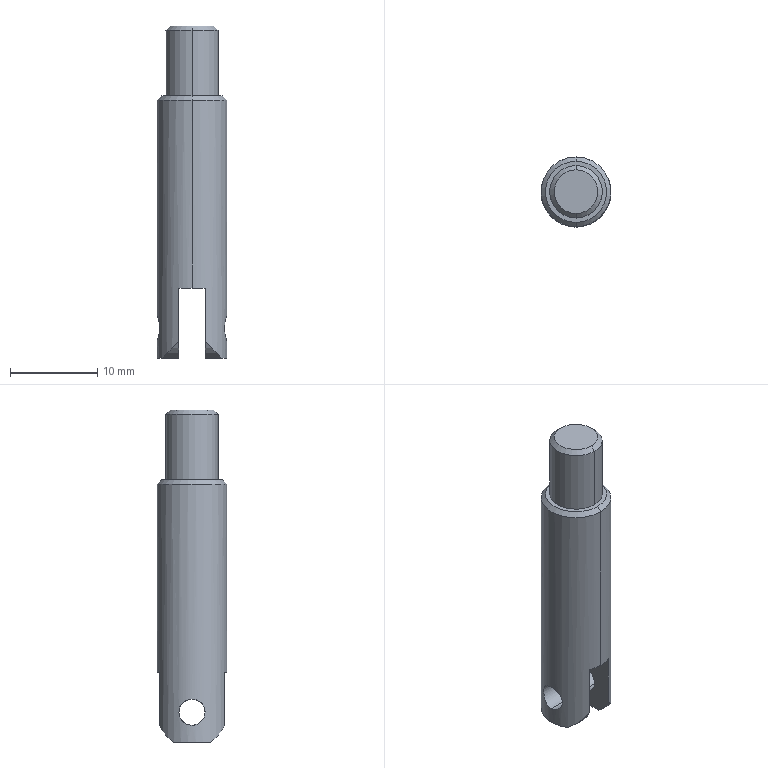Component | SolidWorks | GuideRod1-1 | 1 solid | 23 faces | box 8 x 8 x 38 mm | volume 1503 mm3 | cylinder 12 | plane 7 | cone 4 | commonest cylinder face diameters 8 x6 3 x4 6 x2
build123d program:
from build123d import *

# Parameters (mm, degrees)
SKETCH1_R           = 4
BOSS_EXTRUDE1_DEPTH = 30
SKETCH2_R           = 3
BOSS_EXTRUDE2_DEPTH = 8
CUT_EXTRUDE1_DEPTH  = 13
SKETCH5_W           = 16
SKETCH5_H           = 3
CUT_EXTRUDE2_DEPTH  = 13
SKETCH6_R           = 1.5
CUT_EXTRUDE3_DEPTH  = 13
CHAMFER1_SIZE       = 0.5


with BuildPart() as part:
    # Sketch1 → Boss-Extrude1 (new body)
    with BuildSketch(Plane.XY):
        Circle(SKETCH1_R)
    extrude(amount=BOSS_EXTRUDE1_DEPTH)

    # Sketch2 → Boss-Extrude2 (add)
    with BuildSketch(Plane(origin=(0, 0, 0), x_dir=(-1, 0, 0), z_dir=(0, 0, -1))):
        with Locations(Location((0, 0, 0), (0, 0, 180))):
            Circle(SKETCH2_R)
    extrude(amount=BOSS_EXTRUDE2_DEPTH)

    # Sketch4 → Cut-Extrude1 (cut, symmetric)
    with BuildSketch(Plane(origin=(0, 0, 0), x_dir=(1, 0, 0), z_dir=(0, 1, 0))):
        with BuildLine():
            Line((-4, -26.584), (-9.687, -26.584))
            Line((-9.687, -26.584), (-6.844, -32.06))
            Line((-6.844, -32.06), (5.728, -32.06))
            Line((5.728, -32.06), (7.666, -26.584))
            Line((7.666, -26.584), (4, -26.584))
            ThreePointArc((4, -26.584), (0, -30.584), (-4, -26.584))
        make_face()
    extrude(amount=CUT_EXTRUDE1_DEPTH, both=True, mode=Mode.SUBTRACT)

    # Sketch5 → Cut-Extrude2 (cut, symmetric)
    with BuildSketch(Plane(origin=(0, 0, 0), x_dir=(0, 0, -1), z_dir=(1, 0, 0))):
        with Locations((-30, 0)):
            Rectangle(SKETCH5_W, SKETCH5_H)
    extrude(amount=CUT_EXTRUDE2_DEPTH, both=True, mode=Mode.SUBTRACT)

    # Sketch6 → Cut-Extrude3 (cut, symmetric)
    with BuildSketch(Plane(origin=(0, 0, 0), x_dir=(1, 0, 0), z_dir=(0, 1, 0))):
        with Locations(Location((0, -26.584, 0), (0, 0, 270))):
            Circle(SKETCH6_R)
    extrude(amount=CUT_EXTRUDE3_DEPTH, both=True, mode=Mode.SUBTRACT)

    # Chamfer1
    chamfer1_edges = [part.edges().sort_by_distance(p)[0] for p in [
        (-4, 0, 0),
        (-3, 0, -8),
    ]]
    chamfer(chamfer1_edges, length=CHAMFER1_SIZE)


solid = part.part

# Placed as in the assembly
solid = solid.moved(Location((-15.928, -1.7, 62), (180, 0, -90)))
STEP:
#1=COLOUR_RGB('',0.7922,0.8196,0.9333);
#2=FILL_AREA_STYLE_COLOUR('',#1);
#3=FILL_AREA_STYLE('',(#2));
#4=SURFACE_STYLE_FILL_AREA(#3);
#5=SURFACE_SIDE_STYLE('',(#4));
#6=SURFACE_STYLE_USAGE(.BOTH.,#5);
#7=PRESENTATION_STYLE_ASSIGNMENT((#6));
#8=CARTESIAN_POINT('',(-0.6271,-0.1654,2.756));
#9=VERTEX_POINT('',#8);
#10=CARTESIAN_POINT('',(-0.6271,0.03149,2.756));
#11=VERTEX_POINT('',#10);
#12=CARTESIAN_POINT('',(-0.6271,-0.06694,2.756));
#13=DIRECTION('',(0.,0.,1.));
#14=DIRECTION('',(0.,-1.,0.));
#15=AXIS2_PLACEMENT_3D('',#12,#13,#14);
#16=CIRCLE('',#15,0.09843);
#17=EDGE_CURVE('',#9,#11,#16,.T.);
#18=ORIENTED_EDGE('',*,*,#17,.F.);
#19=CARTESIAN_POINT('',(-0.6271,-0.185,2.736));
#20=VERTEX_POINT('',#19);
#21=CARTESIAN_POINT('',(-0.6271,-0.1654,2.756));
#22=DIRECTION('',(0.,-0.7071,-0.7071));
#23=VECTOR('',#22,39.37);
#24=LINE('',#21,#23);
#25=EDGE_CURVE('',#9,#20,#24,.T.);
#26=ORIENTED_EDGE('',*,*,#25,.T.);
#27=CARTESIAN_POINT('',(-0.6271,0.05117,2.736));
#28=VERTEX_POINT('',#27);
#29=CARTESIAN_POINT('',(-0.6271,-0.06694,2.736));
#30=DIRECTION('',(0.,0.,-1.));
#31=DIRECTION('',(0.,-1.,0.));
#32=AXIS2_PLACEMENT_3D('',#29,#30,#31);
#33=CIRCLE('',#32,0.1181);
#34=EDGE_CURVE('',#28,#20,#33,.T.);
#35=ORIENTED_EDGE('',*,*,#34,.F.);
#36=CARTESIAN_POINT('',(-0.6271,0.03149,2.756));
#37=DIRECTION('',(-0.,0.7071,-0.7071));
#38=VECTOR('',#37,39.37);
#39=LINE('',#36,#38);
#40=EDGE_CURVE('',#11,#28,#39,.T.);
#41=ORIENTED_EDGE('',*,*,#40,.F.);
#42=EDGE_LOOP('',(#18,#26,#35,#41));
#43=FACE_OUTER_BOUND('',#42,.T.);
#44=CARTESIAN_POINT('',(-0.6271,-0.06694,2.756));
#45=DIRECTION('',(0.,0.,-1.));
#46=DIRECTION('',(0.,1.,0.));
#47=AXIS2_PLACEMENT_3D('',#44,#45,#46);
#48=CONICAL_SURFACE('',#47,0.09843,0.7854);
#49=ADVANCED_FACE('',(#43),#48,.T.);
#50=CARTESIAN_POINT('',(-0.6271,-0.2047,2.441));
#51=VERTEX_POINT('',#50);
#52=CARTESIAN_POINT('',(-0.6271,0.07086,2.441));
#53=VERTEX_POINT('',#52);
#54=CARTESIAN_POINT('',(-0.6271,-0.06694,2.441));
#55=DIRECTION('',(0.,0.,1.));
#56=DIRECTION('',(0.,1.,0.));
#57=AXIS2_PLACEMENT_3D('',#54,#55,#56);
#58=CIRCLE('',#57,0.1378);
#59=EDGE_CURVE('',#51,#53,#58,.T.);
#60=ORIENTED_EDGE('',*,*,#59,.F.);
#61=CARTESIAN_POINT('',(-0.6271,-0.2244,2.421));
#62=VERTEX_POINT('',#61);
#63=CARTESIAN_POINT('',(-0.6271,-0.2244,2.421));
#64=DIRECTION('',(0.,-0.7071,-0.7071));
#65=VECTOR('',#64,39.37);
#66=LINE('',#63,#65);
#67=EDGE_CURVE('',#51,#62,#66,.T.);
#68=ORIENTED_EDGE('',*,*,#67,.T.);
#69=CARTESIAN_POINT('',(-0.6271,0.09054,2.421));
#70=VERTEX_POINT('',#69);
#71=CARTESIAN_POINT('',(-0.6271,-0.06694,2.421));
#72=DIRECTION('',(0.,0.,-1.));
#73=DIRECTION('',(0.,1.,0.));
#74=AXIS2_PLACEMENT_3D('',#71,#72,#73);
#75=CIRCLE('',#74,0.1575);
#76=EDGE_CURVE('',#70,#62,#75,.T.);
#77=ORIENTED_EDGE('',*,*,#76,.F.);
#78=CARTESIAN_POINT('',(-0.6271,0.09054,2.421));
#79=DIRECTION('',(-0.,0.7071,-0.7071));
#80=VECTOR('',#79,39.37);
#81=LINE('',#78,#80);
#82=EDGE_CURVE('',#53,#70,#81,.T.);
#83=ORIENTED_EDGE('',*,*,#82,.F.);
#84=EDGE_LOOP('',(#60,#68,#77,#83));
#85=FACE_OUTER_BOUND('',#84,.T.);
#86=CARTESIAN_POINT('',(-0.6271,-0.06694,2.421));
#87=DIRECTION('',(0.,0.,-1.));
#88=DIRECTION('',(0.,1.,0.));
#89=AXIS2_PLACEMENT_3D('',#86,#87,#88);
#90=CONICAL_SURFACE('',#89,0.1575,0.7854);
#91=ADVANCED_FACE('',(#85),#90,.T.);
#92=CARTESIAN_POINT('',(-0.7846,-0.06694,1.453));
#93=VERTEX_POINT('',#92);
#94=CARTESIAN_POINT('',(-0.7846,-0.06694,1.335));
#95=VERTEX_POINT('',#94);
#96=CARTESIAN_POINT('',(-0.7846,-0.06694,1.453));
#97=CARTESIAN_POINT('',(-0.7846,-0.0747,1.453));
#98=CARTESIAN_POINT('',(-0.784,-0.08253,1.452));
#99=CARTESIAN_POINT('',(-0.7824,-0.09323,1.447));
#100=CARTESIAN_POINT('',(-0.7818,-0.09668,1.445));
#101=CARTESIAN_POINT('',(-0.7804,-0.103,1.441));
#102=CARTESIAN_POINT('',(-0.7797,-0.106,1.439));
#103=CARTESIAN_POINT('',(-0.7774,-0.1142,1.431));
#104=CARTESIAN_POINT('',(-0.7759,-0.1185,1.424));
#105=CARTESIAN_POINT('',(-0.7743,-0.1229,1.413));
#106=CARTESIAN_POINT('',(-0.7738,-0.1241,1.41));
#107=CARTESIAN_POINT('',(-0.7732,-0.1256,1.402));
#108=CARTESIAN_POINT('',(-0.7731,-0.126,1.398));
#109=CARTESIAN_POINT('',(-0.7731,-0.126,1.387));
#110=CARTESIAN_POINT('',(-0.7737,-0.1244,1.379));
#111=CARTESIAN_POINT('',(-0.7759,-0.1185,1.364));
#112=CARTESIAN_POINT('',(-0.7774,-0.1141,1.358));
#113=CARTESIAN_POINT('',(-0.7797,-0.106,1.35));
#114=CARTESIAN_POINT('',(-0.7804,-0.103,1.347));
#115=CARTESIAN_POINT('',(-0.7818,-0.0966,1.343));
#116=CARTESIAN_POINT('',(-0.7824,-0.09323,1.341));
#117=CARTESIAN_POINT('',(-0.784,-0.08247,1.337));
#118=CARTESIAN_POINT('',(-0.7846,-0.07482,1.335));
#119=CARTESIAN_POINT('',(-0.7846,-0.06694,1.335));
#120=B_SPLINE_CURVE_WITH_KNOTS('',3,(#96,#97,#98,#99,#100,#101,#102,#103,#104,#105,#106,#107,#108,#109,#110,#111,#112,#113,#114,#115,#116,#117,#118,#119),.UNSPECIFIED.,.F.,.F.,(4,2,2,2,2,2,2,2,2,2,2,4),(0.004733,0.005325,0.005621,0.005916,0.006508,0.006804,0.0071,0.007691,0.008283,0.008578,0.008874,0.009466),.UNSPECIFIED.);
#121=EDGE_CURVE('',#93,#95,#120,.T.);
#122=ORIENTED_EDGE('',*,*,#121,.F.);
#123=CARTESIAN_POINT('',(-0.6861,-0.06694,1.453));
#124=VERTEX_POINT('',#123);
#125=CARTESIAN_POINT('',(-1.139,-0.06694,1.453));
#126=DIRECTION('',(1.,0.,0.));
#127=VECTOR('',#126,39.37);
#128=LINE('',#125,#127);
#129=EDGE_CURVE('',#93,#124,#128,.T.);
#130=ORIENTED_EDGE('',*,*,#129,.T.);
#131=CARTESIAN_POINT('',(-0.6861,-0.06694,1.335));
#132=VERTEX_POINT('',#131);
#133=CARTESIAN_POINT('',(-0.6861,-0.06694,1.394));
#134=DIRECTION('',(-1.,-0.,0.));
#135=DIRECTION('',(0.,0.,1.));
#136=AXIS2_PLACEMENT_3D('',#133,#134,#135);
#137=CIRCLE('',#136,0.05906);
#138=EDGE_CURVE('',#132,#124,#137,.T.);
#139=ORIENTED_EDGE('',*,*,#138,.F.);
#140=CARTESIAN_POINT('',(-1.139,-0.06694,1.335));
#141=DIRECTION('',(1.,0.,0.));
#142=VECTOR('',#141,39.37);
#143=LINE('',#140,#142);
#144=EDGE_CURVE('',#95,#132,#143,.T.);
#145=ORIENTED_EDGE('',*,*,#144,.F.);
#146=EDGE_LOOP('',(#122,#130,#139,#145));
#147=FACE_OUTER_BOUND('',#146,.T.);
#148=CARTESIAN_POINT('',(-1.139,-0.06694,1.394));
#149=DIRECTION('',(1.,0.,0.));
#150=DIRECTION('',(0.,0.,-1.));
#151=AXIS2_PLACEMENT_3D('',#148,#149,#150);
#152=CYLINDRICAL_SURFACE('',#151,0.05906);
#153=ADVANCED_FACE('',(#147),#152,.F.);
#154=CARTESIAN_POINT('',(-0.568,-0.06694,1.453));
#155=VERTEX_POINT('',#154);
#156=CARTESIAN_POINT('',(-0.568,-0.06694,1.335));
#157=VERTEX_POINT('',#156);
#158=CARTESIAN_POINT('',(-0.568,-0.06694,1.394));
#159=DIRECTION('',(1.,0.,0.));
#160=DIRECTION('',(0.,0.,-1.));
#161=AXIS2_PLACEMENT_3D('',#158,#159,#160);
#162=CIRCLE('',#161,0.05906);
#163=EDGE_CURVE('',#155,#157,#162,.T.);
#164=ORIENTED_EDGE('',*,*,#163,.F.);
#165=CARTESIAN_POINT('',(-0.4696,-0.06694,1.453));
#166=VERTEX_POINT('',#165);
#167=CARTESIAN_POINT('',(-1.139,-0.06694,1.453));
#168=DIRECTION('',(1.,0.,0.));
#169=VECTOR('',#168,39.37);
#170=LINE('',#167,#169);
#171=EDGE_CURVE('',#155,#166,#170,.T.);
#172=ORIENTED_EDGE('',*,*,#171,.T.);
#173=CARTESIAN_POINT('',(-0.4696,-0.06694,1.335));
#174=VERTEX_POINT('',#173);
#175=CARTESIAN_POINT('',(-0.4696,-0.06694,1.335));
#176=CARTESIAN_POINT('',(-0.4696,-0.07088,1.335));
#177=CARTESIAN_POINT('',(-0.4698,-0.07475,1.336));
#178=CARTESIAN_POINT('',(-0.4703,-0.08234,1.337));
#179=CARTESIAN_POINT('',(-0.4707,-0.08612,1.338));
#180=CARTESIAN_POINT('',(-0.4723,-0.09682,1.343));
#181=CARTESIAN_POINT('',(-0.4738,-0.1033,1.347));
#182=CARTESIAN_POINT('',(-0.4767,-0.1141,1.358));
#183=CARTESIAN_POINT('',(-0.4783,-0.1185,1.365));
#184=CARTESIAN_POINT('',(-0.4799,-0.1229,1.375));
#185=CARTESIAN_POINT('',(-0.4803,-0.1241,1.379));
#186=CARTESIAN_POINT('',(-0.4809,-0.1256,1.387));
#187=CARTESIAN_POINT('',(-0.4811,-0.126,1.39));
#188=CARTESIAN_POINT('',(-0.4811,-0.126,1.398));
#189=CARTESIAN_POINT('',(-0.4809,-0.1256,1.402));
#190=CARTESIAN_POINT('',(-0.4803,-0.1241,1.41));
#191=CARTESIAN_POINT('',(-0.4799,-0.1229,1.413));
#192=CARTESIAN_POINT('',(-0.4788,-0.1199,1.421));
#193=CARTESIAN_POINT('',(-0.4781,-0.1181,1.424));
#194=CARTESIAN_POINT('',(-0.4767,-0.1139,1.43));
#195=CARTESIAN_POINT('',(-0.476,-0.1114,1.433));
#196=CARTESIAN_POINT('',(-0.4745,-0.106,1.439));
#197=CARTESIAN_POINT('',(-0.4738,-0.103,1.441));
#198=CARTESIAN_POINT('',(-0.4724,-0.09664,1.446));
#199=CARTESIAN_POINT('',(-0.4718,-0.09319,1.447));
#200=CARTESIAN_POINT('',(-0.4702,-0.08254,1.452));
#201=CARTESIAN_POINT('',(-0.4696,-0.0747,1.453));
#202=CARTESIAN_POINT('',(-0.4696,-0.06694,1.453));
#203=B_SPLINE_CURVE_WITH_KNOTS('',3,(#175,#176,#177,#178,#179,#180,#181,#182,#183,#184,#185,#186,#187,#188,#189,#190,#191,#192,#193,#194,#195,#196,#197,#198,#199,#200,#201,#202),.UNSPECIFIED.,.F.,.F.,(4,2,2,2,2,2,2,2,2,2,2,2,2,4),(0.,0.0002958,0.0005917,0.001183,0.001775,0.002071,0.002367,0.002663,0.002958,0.003254,0.00355,0.003846,0.004142,0.004733),.UNSPECIFIED.);
#204=EDGE_CURVE('',#174,#166,#203,.T.);
#205=ORIENTED_EDGE('',*,*,#204,.F.);
#206=CARTESIAN_POINT('',(-1.139,-0.06694,1.335));
#207=DIRECTION('',(1.,0.,0.));
#208=VECTOR('',#207,39.37);
#209=LINE('',#206,#208);
#210=EDGE_CURVE('',#157,#174,#209,.T.);
#211=ORIENTED_EDGE('',*,*,#210,.F.);
#212=EDGE_LOOP('',(#164,#172,#205,#211));
#213=FACE_OUTER_BOUND('',#212,.T.);
#214=CARTESIAN_POINT('',(-1.139,-0.06694,1.394));
#215=DIRECTION('',(1.,0.,0.));
#216=DIRECTION('',(0.,0.,-1.));
#217=AXIS2_PLACEMENT_3D('',#214,#215,#216);
#218=CYLINDRICAL_SURFACE('',#217,0.05906);
#219=ADVANCED_FACE('',(#213),#218,.F.);
#220=ORIENTED_EDGE('',*,*,#34,.T.);
#221=CARTESIAN_POINT('',(-0.6271,-0.185,2.441));
#222=VERTEX_POINT('',#221);
#223=CARTESIAN_POINT('',(-0.6271,-0.185,2.756));
#224=DIRECTION('',(0.,0.,-1.));
#225=VECTOR('',#224,39.37);
#226=LINE('',#223,#225);
#227=EDGE_CURVE('',#20,#222,#226,.T.);
#228=ORIENTED_EDGE('',*,*,#227,.T.);
#229=CARTESIAN_POINT('',(-0.6271,0.05117,2.441));
#230=VERTEX_POINT('',#229);
#231=CARTESIAN_POINT('',(-0.6271,-0.06694,2.441));
#232=DIRECTION('',(0.,0.,1.));
#233=DIRECTION('',(0.,1.,0.));
#234=AXIS2_PLACEMENT_3D('',#231,#232,#233);
#235=CIRCLE('',#234,0.1181);
#236=EDGE_CURVE('',#222,#230,#235,.T.);
#237=ORIENTED_EDGE('',*,*,#236,.T.);
#238=CARTESIAN_POINT('',(-0.6271,0.05117,2.756));
#239=DIRECTION('',(0.,0.,-1.));
#240=VECTOR('',#239,39.37);
#241=LINE('',#238,#240);
#242=EDGE_CURVE('',#28,#230,#241,.T.);
#243=ORIENTED_EDGE('',*,*,#242,.F.);
#244=EDGE_LOOP('',(#220,#228,#237,#243));
#245=FACE_OUTER_BOUND('',#244,.T.);
#246=CARTESIAN_POINT('',(-0.6271,-0.06694,2.756));
#247=DIRECTION('',(0.,0.,-1.));
#248=DIRECTION('',(0.,1.,0.));
#249=AXIS2_PLACEMENT_3D('',#246,#247,#248);
#250=CYLINDRICAL_SURFACE('',#249,0.1181);
#251=ADVANCED_FACE('',(#245),#250,.T.);
#252=ORIENTED_EDGE('',*,*,#204,.T.);
#253=CARTESIAN_POINT('',(-0.4696,-0.06694,1.453));
#254=CARTESIAN_POINT('',(-0.4696,-0.05918,1.453));
#255=CARTESIAN_POINT('',(-0.4702,-0.05135,1.452));
#256=CARTESIAN_POINT('',(-0.4718,-0.04064,1.447));
#257=CARTESIAN_POINT('',(-0.4724,-0.03719,1.445));
#258=CARTESIAN_POINT('',(-0.4738,-0.03083,1.441));
#259=CARTESIAN_POINT('',(-0.4745,-0.02788,1.439));
#260=CARTESIAN_POINT('',(-0.4768,-0.01969,1.431));
#261=CARTESIAN_POINT('',(-0.4783,-0.01538,1.424));
#262=CARTESIAN_POINT('',(-0.4799,-0.01092,1.413));
#263=CARTESIAN_POINT('',(-0.4803,-0.009799,1.41));
#264=CARTESIAN_POINT('',(-0.4809,-0.008273,1.402));
#265=CARTESIAN_POINT('',(-0.4811,-0.00788,1.398));
#266=CARTESIAN_POINT('',(-0.4811,-0.007885,1.387));
#267=CARTESIAN_POINT('',(-0.4804,-0.009469,1.379));
#268=CARTESIAN_POINT('',(-0.4782,-0.0154,1.364));
#269=CARTESIAN_POINT('',(-0.4767,-0.01977,1.358));
#270=CARTESIAN_POINT('',(-0.4745,-0.0279,1.35));
#271=CARTESIAN_POINT('',(-0.4737,-0.03091,1.347));
#272=CARTESIAN_POINT('',(-0.4724,-0.03727,1.343));
#273=CARTESIAN_POINT('',(-0.4718,-0.04065,1.341));
#274=CARTESIAN_POINT('',(-0.4702,-0.05141,1.337));
#275=CARTESIAN_POINT('',(-0.4696,-0.05906,1.335));
#276=CARTESIAN_POINT('',(-0.4696,-0.06694,1.335));
#277=B_SPLINE_CURVE_WITH_KNOTS('',3,(#253,#254,#255,#256,#257,#258,#259,#260,#261,#262,#263,#264,#265,#266,#267,#268,#269,#270,#271,#272,#273,#274,#275,#276),.UNSPECIFIED.,.F.,.F.,(4,2,2,2,2,2,2,2,2,2,2,4),(0.004733,0.005325,0.005621,0.005916,0.006508,0.006804,0.0071,0.007691,0.008283,0.008578,0.008874,0.009466),.UNSPECIFIED.);
#278=EDGE_CURVE('',#166,#174,#277,.T.);
#279=ORIENTED_EDGE('',*,*,#278,.T.);
#280=EDGE_LOOP('',(#252,#279));
#281=FACE_BOUND('',#280,.T.);
#282=CARTESIAN_POINT('',(-0.568,0.07905,1.575));
#283=VERTEX_POINT('',#282);
#284=CARTESIAN_POINT('',(-0.6271,0.09054,1.575));
#285=VERTEX_POINT('',#284);
#286=CARTESIAN_POINT('',(-0.6271,-0.06694,1.575));
#287=DIRECTION('',(0.,0.,1.));
#288=DIRECTION('',(0.,-1.,0.));
#289=AXIS2_PLACEMENT_3D('',#286,#287,#288);
#290=CIRCLE('',#289,0.1575);
#291=EDGE_CURVE('',#283,#285,#290,.T.);
#292=ORIENTED_EDGE('',*,*,#291,.T.);
#293=CARTESIAN_POINT('',(-0.6271,0.09054,1.26));
#294=DIRECTION('',(0.,0.,1.));
#295=VECTOR('',#294,39.37);
#296=LINE('',#293,#295);
#297=EDGE_CURVE('',#285,#70,#296,.T.);
#298=ORIENTED_EDGE('',*,*,#297,.T.);
#299=ORIENTED_EDGE('',*,*,#76,.T.);
#300=CARTESIAN_POINT('',(-0.6271,-0.2244,1.575));
#301=VERTEX_POINT('',#300);
#302=CARTESIAN_POINT('',(-0.6271,-0.2244,1.26));
#303=DIRECTION('',(0.,0.,1.));
#304=VECTOR('',#303,39.37);
#305=LINE('',#302,#304);
#306=EDGE_CURVE('',#301,#62,#305,.T.);
#307=ORIENTED_EDGE('',*,*,#306,.F.);
#308=CARTESIAN_POINT('',(-0.568,-0.2129,1.575));
#309=VERTEX_POINT('',#308);
#310=CARTESIAN_POINT('',(-0.6271,-0.06694,1.575));
#311=DIRECTION('',(0.,0.,1.));
#312=DIRECTION('',(0.,-1.,0.));
#313=AXIS2_PLACEMENT_3D('',#310,#311,#312);
#314=CIRCLE('',#313,0.1575);
#315=EDGE_CURVE('',#301,#309,#314,.T.);
#316=ORIENTED_EDGE('',*,*,#315,.T.);
#317=CARTESIAN_POINT('',(-0.568,-0.2129,1.335));
#318=VERTEX_POINT('',#317);
#319=CARTESIAN_POINT('',(-0.568,-0.2129,1.26));
#320=DIRECTION('',(0.,0.,-1.));
#321=VECTOR('',#320,39.37);
#322=LINE('',#319,#321);
#323=EDGE_CURVE('',#309,#318,#322,.T.);
#324=ORIENTED_EDGE('',*,*,#323,.T.);
#325=CARTESIAN_POINT('',(-0.4926,-0.1489,1.26));
#326=VERTEX_POINT('',#325);
#327=CARTESIAN_POINT('',(-0.568,-0.2129,1.335));
#328=CARTESIAN_POINT('',(-0.5364,-0.2001,1.304));
#329=CARTESIAN_POINT('',(-0.5104,-0.178,1.278));
#330=CARTESIAN_POINT('',(-0.4926,-0.1489,1.26));
#331=(BOUNDED_CURVE()B_SPLINE_CURVE(3,(#327,#328,#329,#330),.UNSPECIFIED.,.F.,.F.)B_SPLINE_CURVE_WITH_KNOTS((4,4),(1.955,2.594),.UNSPECIFIED.)CURVE()GEOMETRIC_REPRESENTATION_ITEM()RATIONAL_B_SPLINE_CURVE((1.,0.9662,0.9662,1.))REPRESENTATION_ITEM(''));
#332=EDGE_CURVE('',#318,#326,#331,.T.);
#333=ORIENTED_EDGE('',*,*,#332,.T.);
#334=CARTESIAN_POINT('',(-0.4926,0.015,1.26));
#335=VERTEX_POINT('',#334);
#336=CARTESIAN_POINT('',(-0.6271,-0.06694,1.26));
#337=DIRECTION('',(0.,0.,-1.));
#338=DIRECTION('',(0.,1.,0.));
#339=AXIS2_PLACEMENT_3D('',#336,#337,#338);
#340=CIRCLE('',#339,0.1575);
#341=EDGE_CURVE('',#335,#326,#340,.T.);
#342=ORIENTED_EDGE('',*,*,#341,.F.);
#343=CARTESIAN_POINT('',(-0.568,0.07905,1.335));
#344=VERTEX_POINT('',#343);
#345=CARTESIAN_POINT('',(-0.4926,0.015,1.26));
#346=CARTESIAN_POINT('',(-0.5104,0.04416,1.278));
#347=CARTESIAN_POINT('',(-0.5364,0.06625,1.304));
#348=CARTESIAN_POINT('',(-0.568,0.07905,1.335));
#349=(BOUNDED_CURVE()B_SPLINE_CURVE(3,(#345,#346,#347,#348),.UNSPECIFIED.,.F.,.F.)B_SPLINE_CURVE_WITH_KNOTS((4,4),(3.689,4.328),.UNSPECIFIED.)CURVE()GEOMETRIC_REPRESENTATION_ITEM()RATIONAL_B_SPLINE_CURVE((1.,0.9662,0.9662,1.))REPRESENTATION_ITEM(''));
#350=EDGE_CURVE('',#335,#344,#349,.T.);
#351=ORIENTED_EDGE('',*,*,#350,.T.);
#352=CARTESIAN_POINT('',(-0.568,0.07905,1.26));
#353=DIRECTION('',(0.,0.,1.));
#354=VECTOR('',#353,39.37);
#355=LINE('',#352,#354);
#356=EDGE_CURVE('',#344,#283,#355,.T.);
#357=ORIENTED_EDGE('',*,*,#356,.T.);
#358=EDGE_LOOP('',(#292,#298,#299,#307,#316,#324,#333,#342,#351,#357));
#359=FACE_OUTER_BOUND('',#358,.T.);
#360=CARTESIAN_POINT('',(-0.6271,-0.06694,1.26));
#361=DIRECTION('',(0.,0.,1.));
#362=DIRECTION('',(0.,-1.,0.));
#363=AXIS2_PLACEMENT_3D('',#360,#361,#362);
#364=CYLINDRICAL_SURFACE('',#363,0.1575);
#365=ADVANCED_FACE('',(#281,#359),#364,.T.);
#366=CARTESIAN_POINT('',(-0.6861,-0.1489,1.26));
#367=VERTEX_POINT('',#366);
#368=CARTESIAN_POINT('',(-0.6861,0.015,1.26));
#369=VERTEX_POINT('',#368);
#370=CARTESIAN_POINT('',(-0.6861,-0.06694,1.26));
#371=DIRECTION('',(-0.,1.,0.));
#372=VECTOR('',#371,39.37);
#373=LINE('',#370,#372);
#374=EDGE_CURVE('',#367,#369,#373,.T.);
#375=ORIENTED_EDGE('',*,*,#374,.F.);
#376=CARTESIAN_POINT('',(-0.7616,-0.1489,1.26));
#377=VERTEX_POINT('',#376);
#378=CARTESIAN_POINT('',(-1.139,-0.1489,1.26));
#379=DIRECTION('',(1.,0.,0.));
#380=VECTOR('',#379,39.37);
#381=LINE('',#378,#380);
#382=EDGE_CURVE('',#377,#367,#381,.T.);
#383=ORIENTED_EDGE('',*,*,#382,.F.);
#384=CARTESIAN_POINT('',(-0.7616,0.015,1.26));
#385=VERTEX_POINT('',#384);
#386=CARTESIAN_POINT('',(-0.6271,-0.06694,1.26));
#387=DIRECTION('',(0.,0.,-1.));
#388=DIRECTION('',(0.,1.,0.));
#389=AXIS2_PLACEMENT_3D('',#386,#387,#388);
#390=CIRCLE('',#389,0.1575);
#391=EDGE_CURVE('',#377,#385,#390,.T.);
#392=ORIENTED_EDGE('',*,*,#391,.T.);
#393=CARTESIAN_POINT('',(-1.139,0.015,1.26));
#394=DIRECTION('',(-1.,-0.,0.));
#395=VECTOR('',#394,39.37);
#396=LINE('',#393,#395);
#397=EDGE_CURVE('',#369,#385,#396,.T.);
#398=ORIENTED_EDGE('',*,*,#397,.F.);
#399=EDGE_LOOP('',(#375,#383,#392,#398));
#400=FACE_OUTER_BOUND('',#399,.T.);
#401=CARTESIAN_POINT('',(-0.6271,-0.06694,1.26));
#402=DIRECTION('',(0.,0.,-1.));
#403=DIRECTION('',(-0.,1.,0.));
#404=AXIS2_PLACEMENT_3D('',#401,#402,#403);
#405=PLANE('',#404);
#406=ADVANCED_FACE('',(#400),#405,.T.);
#407=ORIENTED_EDGE('',*,*,#382,.T.);
#408=CARTESIAN_POINT('',(-0.6861,-0.2129,1.335));
#409=VERTEX_POINT('',#408);
#410=CARTESIAN_POINT('',(-0.6861,-0.06694,1.394));
#411=DIRECTION('',(-1.,-0.,0.));
#412=DIRECTION('',(0.,0.,1.));
#413=AXIS2_PLACEMENT_3D('',#410,#411,#412);
#414=CIRCLE('',#413,0.1575);
#415=EDGE_CURVE('',#367,#409,#414,.T.);
#416=ORIENTED_EDGE('',*,*,#415,.T.);
#417=CARTESIAN_POINT('',(-0.7616,-0.1489,1.26));
#418=CARTESIAN_POINT('',(-0.7438,-0.178,1.278));
#419=CARTESIAN_POINT('',(-0.7178,-0.2001,1.304));
#420=CARTESIAN_POINT('',(-0.6861,-0.2129,1.335));
#421=(BOUNDED_CURVE()B_SPLINE_CURVE(3,(#417,#418,#419,#420),.UNSPECIFIED.,.F.,.F.)B_SPLINE_CURVE_WITH_KNOTS((4,4),(3.689,4.328),.UNSPECIFIED.)CURVE()GEOMETRIC_REPRESENTATION_ITEM()RATIONAL_B_SPLINE_CURVE((1.,0.9662,0.9662,1.))REPRESENTATION_ITEM(''));
#422=EDGE_CURVE('',#377,#409,#421,.T.);
#423=ORIENTED_EDGE('',*,*,#422,.F.);
#424=EDGE_LOOP('',(#407,#416,#423));
#425=FACE_OUTER_BOUND('',#424,.T.);
#426=CARTESIAN_POINT('',(-1.139,-0.06694,1.394));
#427=DIRECTION('',(1.,0.,0.));
#428=DIRECTION('',(0.,0.,-1.));
#429=AXIS2_PLACEMENT_3D('',#426,#427,#428);
#430=CYLINDRICAL_SURFACE('',#429,0.1575);
#431=ADVANCED_FACE('',(#425),#430,.T.);
#432=CARTESIAN_POINT('',(-0.6861,0.07905,1.335));
#433=VERTEX_POINT('',#432);
#434=CARTESIAN_POINT('',(-0.6861,0.07905,1.335));
#435=CARTESIAN_POINT('',(-0.7178,0.06625,1.304));
#436=CARTESIAN_POINT('',(-0.7438,0.04416,1.278));
#437=CARTESIAN_POINT('',(-0.7616,0.015,1.26));
#438=(BOUNDED_CURVE()B_SPLINE_CURVE(3,(#434,#435,#436,#437),.UNSPECIFIED.,.F.,.T.)B_SPLINE_CURVE_WITH_KNOTS((4,4),(1.955,2.594),.UNSPECIFIED.)CURVE()GEOMETRIC_REPRESENTATION_ITEM()RATIONAL_B_SPLINE_CURVE((1.,0.9662,0.9662,1.))REPRESENTATION_ITEM(''));
#439=EDGE_CURVE('',#433,#385,#438,.T.);
#440=ORIENTED_EDGE('',*,*,#439,.F.);
#441=CARTESIAN_POINT('',(-0.6861,-0.06694,1.394));
#442=DIRECTION('',(-1.,-0.,0.));
#443=DIRECTION('',(0.,0.,1.));
#444=AXIS2_PLACEMENT_3D('',#441,#442,#443);
#445=CIRCLE('',#444,0.1575);
#446=EDGE_CURVE('',#433,#369,#445,.T.);
#447=ORIENTED_EDGE('',*,*,#446,.T.);
#448=ORIENTED_EDGE('',*,*,#397,.T.);
#449=EDGE_LOOP('',(#440,#447,#448));
#450=FACE_OUTER_BOUND('',#449,.T.);
#451=CARTESIAN_POINT('',(-1.139,-0.06694,1.394));
#452=DIRECTION('',(1.,0.,0.));
#453=DIRECTION('',(0.,0.,-1.));
#454=AXIS2_PLACEMENT_3D('',#451,#452,#453);
#455=CYLINDRICAL_SURFACE('',#454,0.1575);
#456=ADVANCED_FACE('',(#450),#455,.T.);
#457=CARTESIAN_POINT('',(-0.6271,-0.06694,2.441));
#458=DIRECTION('',(0.,0.,1.));
#459=DIRECTION('',(0.,1.,0.));
#460=AXIS2_PLACEMENT_3D('',#457,#458,#459);
#461=CIRCLE('',#460,0.1378);
#462=EDGE_CURVE('',#53,#51,#461,.T.);
#463=ORIENTED_EDGE('',*,*,#462,.T.);
#464=ORIENTED_EDGE('',*,*,#59,.T.);
#465=EDGE_LOOP('',(#463,#464));
#466=FACE_OUTER_BOUND('',#465,.T.);
#467=CARTESIAN_POINT('',(-0.6271,-0.06694,2.441));
#468=DIRECTION('',(0.,0.,1.));
#469=DIRECTION('',(0.,1.,0.));
#470=AXIS2_PLACEMENT_3D('',#467,#468,#469);
#471=CIRCLE('',#470,0.1181);
#472=EDGE_CURVE('',#230,#222,#471,.T.);
#473=ORIENTED_EDGE('',*,*,#472,.F.);
#474=ORIENTED_EDGE('',*,*,#236,.F.);
#475=EDGE_LOOP('',(#473,#474));
#476=FACE_BOUND('',#475,.T.);
#477=CARTESIAN_POINT('',(-0.6271,-0.06694,2.441));
#478=DIRECTION('',(0.,0.,-1.));
#479=DIRECTION('',(-0.,1.,0.));
#480=AXIS2_PLACEMENT_3D('',#477,#478,#479);
#481=PLANE('',#480);
#482=ADVANCED_FACE('',(#466,#476),#481,.F.);
#483=ORIENTED_EDGE('',*,*,#297,.F.);
#484=CARTESIAN_POINT('',(-0.6861,0.07905,1.575));
#485=VERTEX_POINT('',#484);
#486=CARTESIAN_POINT('',(-0.6271,-0.06694,1.575));
#487=DIRECTION('',(0.,0.,1.));
#488=DIRECTION('',(0.,-1.,0.));
#489=AXIS2_PLACEMENT_3D('',#486,#487,#488);
#490=CIRCLE('',#489,0.1575);
#491=EDGE_CURVE('',#285,#485,#490,.T.);
#492=ORIENTED_EDGE('',*,*,#491,.T.);
#493=CARTESIAN_POINT('',(-0.6861,0.07905,1.26));
#494=DIRECTION('',(0.,0.,-1.));
#495=VECTOR('',#494,39.37);
#496=LINE('',#493,#495);
#497=EDGE_CURVE('',#485,#433,#496,.T.);
#498=ORIENTED_EDGE('',*,*,#497,.T.);
#499=ORIENTED_EDGE('',*,*,#439,.T.);
#500=ORIENTED_EDGE('',*,*,#391,.F.);
#501=ORIENTED_EDGE('',*,*,#422,.T.);
#502=CARTESIAN_POINT('',(-0.6861,-0.2129,1.575));
#503=VERTEX_POINT('',#502);
#504=CARTESIAN_POINT('',(-0.6861,-0.2129,1.26));
#505=DIRECTION('',(0.,0.,1.));
#506=VECTOR('',#505,39.37);
#507=LINE('',#504,#506);
#508=EDGE_CURVE('',#409,#503,#507,.T.);
#509=ORIENTED_EDGE('',*,*,#508,.T.);
#510=CARTESIAN_POINT('',(-0.6271,-0.06694,1.575));
#511=DIRECTION('',(0.,0.,1.));
#512=DIRECTION('',(0.,-1.,0.));
#513=AXIS2_PLACEMENT_3D('',#510,#511,#512);
#514=CIRCLE('',#513,0.1575);
#515=EDGE_CURVE('',#503,#301,#514,.T.);
#516=ORIENTED_EDGE('',*,*,#515,.T.);
#517=ORIENTED_EDGE('',*,*,#306,.T.);
#518=CARTESIAN_POINT('',(-0.6271,-0.06694,2.421));
#519=DIRECTION('',(0.,0.,-1.));
#520=DIRECTION('',(0.,1.,0.));
#521=AXIS2_PLACEMENT_3D('',#518,#519,#520);
#522=CIRCLE('',#521,0.1575);
#523=EDGE_CURVE('',#62,#70,#522,.T.);
#524=ORIENTED_EDGE('',*,*,#523,.T.);
#525=EDGE_LOOP('',(#483,#492,#498,#499,#500,#501,#509,#516,#517,#524));
#526=FACE_OUTER_BOUND('',#525,.T.);
#527=CARTESIAN_POINT('',(-0.7846,-0.06694,1.335));
#528=CARTESIAN_POINT('',(-0.7846,-0.063,1.335));
#529=CARTESIAN_POINT('',(-0.7844,-0.05913,1.336));
#530=CARTESIAN_POINT('',(-0.7839,-0.05153,1.337));
#531=CARTESIAN_POINT('',(-0.7834,-0.04776,1.338));
#532=CARTESIAN_POINT('',(-0.7819,-0.03705,1.343));
#533=CARTESIAN_POINT('',(-0.7804,-0.03055,1.347));
#534=CARTESIAN_POINT('',(-0.7774,-0.01976,1.358));
#535=CARTESIAN_POINT('',(-0.7759,-0.01538,1.365));
#536=CARTESIAN_POINT('',(-0.7743,-0.01095,1.375));
#537=CARTESIAN_POINT('',(-0.7738,-0.009798,1.379));
#538=CARTESIAN_POINT('',(-0.7732,-0.008267,1.387));
#539=CARTESIAN_POINT('',(-0.7731,-0.007883,1.39));
#540=CARTESIAN_POINT('',(-0.7731,-0.007879,1.398));
#541=CARTESIAN_POINT('',(-0.7732,-0.008272,1.402));
#542=CARTESIAN_POINT('',(-0.7738,-0.009798,1.41));
#543=CARTESIAN_POINT('',(-0.7743,-0.01093,1.413));
#544=CARTESIAN_POINT('',(-0.7754,-0.01393,1.421));
#545=CARTESIAN_POINT('',(-0.776,-0.01575,1.424));
#546=CARTESIAN_POINT('',(-0.7774,-0.02001,1.43));
#547=CARTESIAN_POINT('',(-0.7782,-0.02249,1.433));
#548=CARTESIAN_POINT('',(-0.7797,-0.0279,1.439));
#549=CARTESIAN_POINT('',(-0.7804,-0.03085,1.441));
#550=CARTESIAN_POINT('',(-0.7818,-0.03723,1.446));
#551=CARTESIAN_POINT('',(-0.7824,-0.04068,1.447));
#552=CARTESIAN_POINT('',(-0.784,-0.05134,1.452));
#553=CARTESIAN_POINT('',(-0.7846,-0.05917,1.453));
#554=CARTESIAN_POINT('',(-0.7846,-0.06694,1.453));
#555=B_SPLINE_CURVE_WITH_KNOTS('',3,(#527,#528,#529,#530,#531,#532,#533,#534,#535,#536,#537,#538,#539,#540,#541,#542,#543,#544,#545,#546,#547,#548,#549,#550,#551,#552,#553,#554),.UNSPECIFIED.,.F.,.F.,(4,2,2,2,2,2,2,2,2,2,2,2,2,4),(0.,0.0002958,0.0005917,0.001183,0.001775,0.002071,0.002367,0.002663,0.002958,0.003254,0.00355,0.003846,0.004142,0.004733),.UNSPECIFIED.);
#556=EDGE_CURVE('',#95,#93,#555,.T.);
#557=ORIENTED_EDGE('',*,*,#556,.T.);
#558=ORIENTED_EDGE('',*,*,#121,.T.);
#559=EDGE_LOOP('',(#557,#558));
#560=FACE_BOUND('',#559,.T.);
#561=CARTESIAN_POINT('',(-0.6271,-0.06694,1.26));
#562=DIRECTION('',(0.,0.,1.));
#563=DIRECTION('',(0.,-1.,0.));
#564=AXIS2_PLACEMENT_3D('',#561,#562,#563);
#565=CYLINDRICAL_SURFACE('',#564,0.1575);
#566=ADVANCED_FACE('',(#526,#560),#565,.T.);
#567=CARTESIAN_POINT('',(-0.568,0.015,1.26));
#568=VERTEX_POINT('',#567);
#569=CARTESIAN_POINT('',(-0.568,-0.1489,1.26));
#570=VERTEX_POINT('',#569);
#571=CARTESIAN_POINT('',(-0.568,-0.06694,1.26));
#572=DIRECTION('',(0.,-1.,0.));
#573=VECTOR('',#572,39.37);
#574=LINE('',#571,#573);
#575=EDGE_CURVE('',#568,#570,#574,.T.);
#576=ORIENTED_EDGE('',*,*,#575,.F.);
#577=CARTESIAN_POINT('',(-1.139,0.015,1.26));
#578=DIRECTION('',(-1.,-0.,0.));
#579=VECTOR('',#578,39.37);
#580=LINE('',#577,#579);
#581=EDGE_CURVE('',#335,#568,#580,.T.);
#582=ORIENTED_EDGE('',*,*,#581,.F.);
#583=ORIENTED_EDGE('',*,*,#341,.T.);
#584=CARTESIAN_POINT('',(-1.139,-0.1489,1.26));
#585=DIRECTION('',(1.,0.,0.));
#586=VECTOR('',#585,39.37);
#587=LINE('',#584,#586);
#588=EDGE_CURVE('',#570,#326,#587,.T.);
#589=ORIENTED_EDGE('',*,*,#588,.F.);
#590=EDGE_LOOP('',(#576,#582,#583,#589));
#591=FACE_OUTER_BOUND('',#590,.T.);
#592=CARTESIAN_POINT('',(-0.6271,-0.06694,1.26));
#593=DIRECTION('',(0.,0.,-1.));
#594=DIRECTION('',(-0.,1.,0.));
#595=AXIS2_PLACEMENT_3D('',#592,#593,#594);
#596=PLANE('',#595);
#597=ADVANCED_FACE('',(#591),#596,.T.);
#598=ORIENTED_EDGE('',*,*,#227,.F.);
#599=CARTESIAN_POINT('',(-0.6271,-0.06694,2.736));
#600=DIRECTION('',(0.,0.,-1.));
#601=DIRECTION('',(0.,-1.,0.));
#602=AXIS2_PLACEMENT_3D('',#599,#600,#601);
#603=CIRCLE('',#602,0.1181);
#604=EDGE_CURVE('',#20,#28,#603,.T.);
#605=ORIENTED_EDGE('',*,*,#604,.T.);
#606=ORIENTED_EDGE('',*,*,#242,.T.);
#607=ORIENTED_EDGE('',*,*,#472,.T.);
#608=EDGE_LOOP('',(#598,#605,#606,#607));
#609=FACE_OUTER_BOUND('',#608,.T.);
#610=CARTESIAN_POINT('',(-0.6271,-0.06694,2.756));
#611=DIRECTION('',(0.,0.,-1.));
#612=DIRECTION('',(0.,1.,0.));
#613=AXIS2_PLACEMENT_3D('',#610,#611,#612);
#614=CYLINDRICAL_SURFACE('',#613,0.1181);
#615=ADVANCED_FACE('',(#609),#614,.T.);
#616=CARTESIAN_POINT('',(-0.6271,-0.06694,2.756));
#617=DIRECTION('',(0.,0.,1.));
#618=DIRECTION('',(0.,-1.,0.));
#619=AXIS2_PLACEMENT_3D('',#616,#617,#618);
#620=CIRCLE('',#619,0.09843);
#621=EDGE_CURVE('',#11,#9,#620,.T.);
#622=ORIENTED_EDGE('',*,*,#621,.T.);
#623=ORIENTED_EDGE('',*,*,#17,.T.);
#624=EDGE_LOOP('',(#622,#623));
#625=FACE_OUTER_BOUND('',#624,.T.);
#626=CARTESIAN_POINT('',(-0.6271,-0.06694,2.756));
#627=DIRECTION('',(0.,0.,1.));
#628=DIRECTION('',(0.,-1.,0.));
#629=AXIS2_PLACEMENT_3D('',#626,#627,#628);
#630=PLANE('',#629);
#631=ADVANCED_FACE('',(#625),#630,.T.);
#632=ORIENTED_EDGE('',*,*,#332,.F.);
#633=CARTESIAN_POINT('',(-0.568,-0.06694,1.394));
#634=DIRECTION('',(1.,0.,0.));
#635=DIRECTION('',(0.,0.,-1.));
#636=AXIS2_PLACEMENT_3D('',#633,#634,#635);
#637=CIRCLE('',#636,0.1575);
#638=EDGE_CURVE('',#318,#570,#637,.T.);
#639=ORIENTED_EDGE('',*,*,#638,.T.);
#640=ORIENTED_EDGE('',*,*,#588,.T.);
#641=EDGE_LOOP('',(#632,#639,#640));
#642=FACE_OUTER_BOUND('',#641,.T.);
#643=CARTESIAN_POINT('',(-1.139,-0.06694,1.394));
#644=DIRECTION('',(1.,0.,0.));
#645=DIRECTION('',(0.,0.,-1.));
#646=AXIS2_PLACEMENT_3D('',#643,#644,#645);
#647=CYLINDRICAL_SURFACE('',#646,0.1575);
#648=ADVANCED_FACE('',(#642),#647,.T.);
#649=ORIENTED_EDGE('',*,*,#581,.T.);
#650=CARTESIAN_POINT('',(-0.568,-0.06694,1.394));
#651=DIRECTION('',(1.,0.,0.));
#652=DIRECTION('',(0.,0.,-1.));
#653=AXIS2_PLACEMENT_3D('',#650,#651,#652);
#654=CIRCLE('',#653,0.1575);
#655=EDGE_CURVE('',#568,#344,#654,.T.);
#656=ORIENTED_EDGE('',*,*,#655,.T.);
#657=ORIENTED_EDGE('',*,*,#350,.F.);
#658=EDGE_LOOP('',(#649,#656,#657));
#659=FACE_OUTER_BOUND('',#658,.T.);
#660=CARTESIAN_POINT('',(-1.139,-0.06694,1.394));
#661=DIRECTION('',(1.,0.,0.));
#662=DIRECTION('',(0.,0.,-1.));
#663=AXIS2_PLACEMENT_3D('',#660,#661,#662);
#664=CYLINDRICAL_SURFACE('',#663,0.1575);
#665=ADVANCED_FACE('',(#659),#664,.T.);
#666=CARTESIAN_POINT('',(-0.568,-0.5787,1.575));
#667=DIRECTION('',(-0.,1.,0.));
#668=VECTOR('',#667,39.37);
#669=LINE('',#666,#668);
#670=EDGE_CURVE('',#309,#283,#669,.T.);
#671=ORIENTED_EDGE('',*,*,#670,.F.);
#672=ORIENTED_EDGE('',*,*,#315,.F.);
#673=ORIENTED_EDGE('',*,*,#515,.F.);
#674=CARTESIAN_POINT('',(-0.6861,-0.5787,1.575));
#675=DIRECTION('',(-0.,1.,0.));
#676=VECTOR('',#675,39.37);
#677=LINE('',#674,#676);
#678=EDGE_CURVE('',#503,#485,#677,.T.);
#679=ORIENTED_EDGE('',*,*,#678,.T.);
#680=ORIENTED_EDGE('',*,*,#491,.F.);
#681=ORIENTED_EDGE('',*,*,#291,.F.);
#682=EDGE_LOOP('',(#671,#672,#673,#679,#680,#681));
#683=FACE_OUTER_BOUND('',#682,.T.);
#684=CARTESIAN_POINT('',(-0.568,-0.5787,1.575));
#685=DIRECTION('',(0.,0.,1.));
#686=DIRECTION('',(0.,-1.,0.));
#687=AXIS2_PLACEMENT_3D('',#684,#685,#686);
#688=PLANE('',#687);
#689=ADVANCED_FACE('',(#683),#688,.F.);
#690=ORIENTED_EDGE('',*,*,#138,.T.);
#691=CARTESIAN_POINT('',(-0.6861,-0.06694,1.394));
#692=DIRECTION('',(-1.,-0.,0.));
#693=DIRECTION('',(0.,0.,1.));
#694=AXIS2_PLACEMENT_3D('',#691,#692,#693);
#695=CIRCLE('',#694,0.05906);
#696=EDGE_CURVE('',#124,#132,#695,.T.);
#697=ORIENTED_EDGE('',*,*,#696,.T.);
#698=EDGE_LOOP('',(#690,#697));
#699=FACE_BOUND('',#698,.T.);
#700=ORIENTED_EDGE('',*,*,#415,.F.);
#701=ORIENTED_EDGE('',*,*,#374,.T.);
#702=ORIENTED_EDGE('',*,*,#446,.F.);
#703=ORIENTED_EDGE('',*,*,#497,.F.);
#704=ORIENTED_EDGE('',*,*,#678,.F.);
#705=ORIENTED_EDGE('',*,*,#508,.F.);
#706=EDGE_LOOP('',(#700,#701,#702,#703,#704,#705));
#707=FACE_OUTER_BOUND('',#706,.T.);
#708=CARTESIAN_POINT('',(-0.6861,-0.5787,0.9449));
#709=DIRECTION('',(-1.,-0.,0.));
#710=DIRECTION('',(0.,0.,1.));
#711=AXIS2_PLACEMENT_3D('',#708,#709,#710);
#712=PLANE('',#711);
#713=ADVANCED_FACE('',(#699,#707),#712,.F.);
#714=CARTESIAN_POINT('',(-0.568,-0.06694,1.394));
#715=DIRECTION('',(1.,0.,0.));
#716=DIRECTION('',(0.,0.,-1.));
#717=AXIS2_PLACEMENT_3D('',#714,#715,#716);
#718=CIRCLE('',#717,0.05906);
#719=EDGE_CURVE('',#157,#155,#718,.T.);
#720=ORIENTED_EDGE('',*,*,#719,.T.);
#721=ORIENTED_EDGE('',*,*,#163,.T.);
#722=EDGE_LOOP('',(#720,#721));
#723=FACE_BOUND('',#722,.T.);
#724=ORIENTED_EDGE('',*,*,#670,.T.);
#725=ORIENTED_EDGE('',*,*,#356,.F.);
#726=ORIENTED_EDGE('',*,*,#655,.F.);
#727=ORIENTED_EDGE('',*,*,#575,.T.);
#728=ORIENTED_EDGE('',*,*,#638,.F.);
#729=ORIENTED_EDGE('',*,*,#323,.F.);
#730=EDGE_LOOP('',(#724,#725,#726,#727,#728,#729));
#731=FACE_OUTER_BOUND('',#730,.T.);
#732=CARTESIAN_POINT('',(-0.568,-0.5787,0.9449));
#733=DIRECTION('',(1.,0.,0.));
#734=DIRECTION('',(0.,0.,-1.));
#735=AXIS2_PLACEMENT_3D('',#732,#733,#734);
#736=PLANE('',#735);
#737=ADVANCED_FACE('',(#723,#731),#736,.F.);
#738=ORIENTED_EDGE('',*,*,#171,.F.);
#739=ORIENTED_EDGE('',*,*,#719,.F.);
#740=ORIENTED_EDGE('',*,*,#210,.T.);
#741=ORIENTED_EDGE('',*,*,#278,.F.);
#742=EDGE_LOOP('',(#738,#739,#740,#741));
#743=FACE_OUTER_BOUND('',#742,.T.);
#744=CARTESIAN_POINT('',(-1.139,-0.06694,1.394));
#745=DIRECTION('',(1.,0.,0.));
#746=DIRECTION('',(0.,0.,-1.));
#747=AXIS2_PLACEMENT_3D('',#744,#745,#746);
#748=CYLINDRICAL_SURFACE('',#747,0.05906);
#749=ADVANCED_FACE('',(#743),#748,.F.);
#750=ORIENTED_EDGE('',*,*,#129,.F.);
#751=ORIENTED_EDGE('',*,*,#556,.F.);
#752=ORIENTED_EDGE('',*,*,#144,.T.);
#753=ORIENTED_EDGE('',*,*,#696,.F.);
#754=EDGE_LOOP('',(#750,#751,#752,#753));
#755=FACE_OUTER_BOUND('',#754,.T.);
#756=CARTESIAN_POINT('',(-1.139,-0.06694,1.394));
#757=DIRECTION('',(1.,0.,0.));
#758=DIRECTION('',(0.,0.,-1.));
#759=AXIS2_PLACEMENT_3D('',#756,#757,#758);
#760=CYLINDRICAL_SURFACE('',#759,0.05906);
#761=ADVANCED_FACE('',(#755),#760,.F.);
#762=ORIENTED_EDGE('',*,*,#67,.F.);
#763=ORIENTED_EDGE('',*,*,#462,.F.);
#764=ORIENTED_EDGE('',*,*,#82,.T.);
#765=ORIENTED_EDGE('',*,*,#523,.F.);
#766=EDGE_LOOP('',(#762,#763,#764,#765));
#767=FACE_OUTER_BOUND('',#766,.T.);
#768=CARTESIAN_POINT('',(-0.6271,-0.06694,2.421));
#769=DIRECTION('',(0.,0.,-1.));
#770=DIRECTION('',(0.,1.,0.));
#771=AXIS2_PLACEMENT_3D('',#768,#769,#770);
#772=CONICAL_SURFACE('',#771,0.1575,0.7854);
#773=ADVANCED_FACE('',(#767),#772,.T.);
#774=ORIENTED_EDGE('',*,*,#25,.F.);
#775=ORIENTED_EDGE('',*,*,#621,.F.);
#776=ORIENTED_EDGE('',*,*,#40,.T.);
#777=ORIENTED_EDGE('',*,*,#604,.F.);
#778=EDGE_LOOP('',(#774,#775,#776,#777));
#779=FACE_OUTER_BOUND('',#778,.T.);
#780=CARTESIAN_POINT('',(-0.6271,-0.06694,2.756));
#781=DIRECTION('',(0.,0.,-1.));
#782=DIRECTION('',(0.,1.,0.));
#783=AXIS2_PLACEMENT_3D('',#780,#781,#782);
#784=CONICAL_SURFACE('',#783,0.09843,0.7854);
#785=ADVANCED_FACE('',(#779),#784,.T.);
#786=CLOSED_SHELL('',(#49,#91,#153,#219,#251,#365,#406,#431,#456,#482,#566,#597,#615,#631,#648,#665,#689,#713,#737,#749,#761,#773,#785));
#787=MANIFOLD_SOLID_BREP('',#786);
#788=STYLED_ITEM('',(#7),#787);
#789=PRESENTATION_LAYER_ASSIGNMENT('','',(#788));
#790=CARTESIAN_POINT('',(0.,0.,0.));
#791=DIRECTION('',(0.,0.,1.));
#792=DIRECTION('',(1.,0.,0.));
#793=AXIS2_PLACEMENT_3D('',#790,#791,#792);
#794=(LENGTH_UNIT()NAMED_UNIT(*)SI_UNIT($,.METRE.));
#795=LENGTH_MEASURE_WITH_UNIT(LENGTH_MEASURE(0.0254),#794);
#796=DIMENSIONAL_EXPONENTS(1.,0.,0.,0.,0.,0.,0.);
#797=(CONVERSION_BASED_UNIT('',#795)LENGTH_UNIT()NAMED_UNIT(#796));
#798=UNCERTAINTY_MEASURE_WITH_UNIT(LENGTH_MEASURE(0.00001),#797,'','');
#799=(NAMED_UNIT(*)PLANE_ANGLE_UNIT()SI_UNIT($,.RADIAN.));
#800=(NAMED_UNIT(*)SI_UNIT($,.STERADIAN.)SOLID_ANGLE_UNIT());
#801=(GEOMETRIC_REPRESENTATION_CONTEXT(3)GLOBAL_UNCERTAINTY_ASSIGNED_CONTEXT((#798))GLOBAL_UNIT_ASSIGNED_CONTEXT((#797,#799,#800))REPRESENTATION_CONTEXT('',''));
#802=ADVANCED_BREP_SHAPE_REPRESENTATION('',(#787,#793),#801);
#803=(LENGTH_UNIT()NAMED_UNIT(*)SI_UNIT($,.METRE.));
#804=LENGTH_MEASURE_WITH_UNIT(LENGTH_MEASURE(0.0254),#803);
#805=DIMENSIONAL_EXPONENTS(1.,0.,0.,0.,0.,0.,0.);
#806=(CONVERSION_BASED_UNIT('',#804)LENGTH_UNIT()NAMED_UNIT(#805));
#807=UNCERTAINTY_MEASURE_WITH_UNIT(LENGTH_MEASURE(0.00001),#806,'','');
#808=(NAMED_UNIT(*)PLANE_ANGLE_UNIT()SI_UNIT($,.RADIAN.));
#809=(NAMED_UNIT(*)SI_UNIT($,.STERADIAN.)SOLID_ANGLE_UNIT());
#810=(GEOMETRIC_REPRESENTATION_CONTEXT(3)GLOBAL_UNCERTAINTY_ASSIGNED_CONTEXT((#807))GLOBAL_UNIT_ASSIGNED_CONTEXT((#806,#808,#809))REPRESENTATION_CONTEXT('',''));
#811=MECHANICAL_DESIGN_GEOMETRIC_PRESENTATION_REPRESENTATION('',(#788),#810);